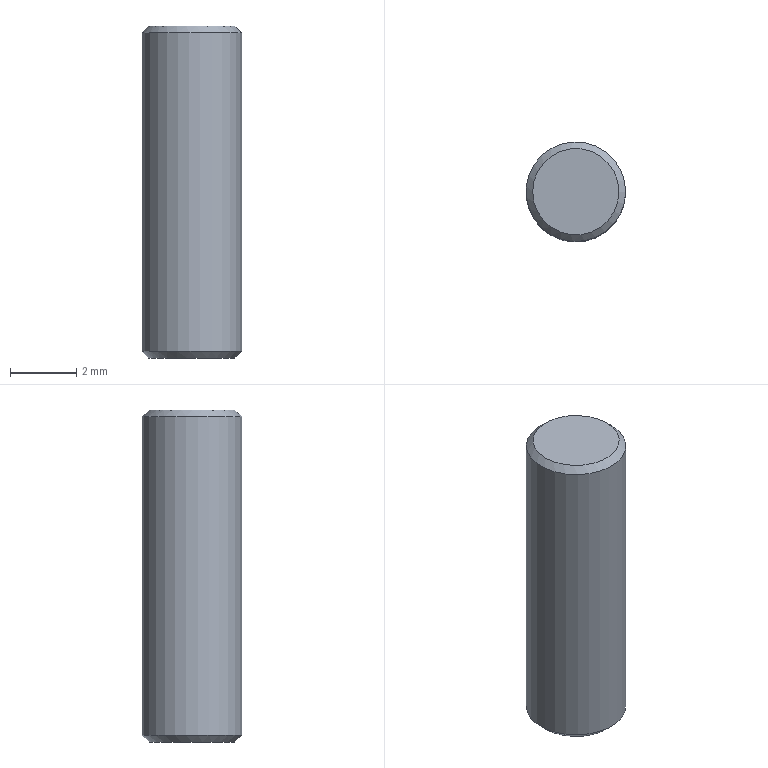Component | NX | GB120-3X10 | 1 solid | 5 faces | box 3 x 3 x 10 mm | volume 70 mm3 | plane 2 | cone 2 | cylinder 1 | commonest cylinder face diameters 3 x1
STEP:
#1=CARTESIAN_POINT('',(0.,0.,0.));
#2=DIRECTION('',(0.,0.,1.));
#3=DIRECTION('',(1.,0.,0.));
#4=AXIS2_PLACEMENT_3D('',#1,#2,#3);
#5=CARTESIAN_POINT('',(-31.5,17.,43.8));
#6=VERTEX_POINT('',#5);
#7=CARTESIAN_POINT('',(-33.,17.,43.8));
#8=DIRECTION('',(0.,0.,-1.));
#9=DIRECTION('',(1.,0.,0.));
#10=AXIS2_PLACEMENT_3D('',#7,#8,#9);
#11=CIRCLE('',#10,1.5);
#12=CARTESIAN_POINT('',(-33.,17.,44.));
#13=DIRECTION('',(0.,0.,-1.));
#14=DIRECTION('',(-1.,0.,0.));
#15=AXIS2_PLACEMENT_3D('',#12,#13,#14);
#16=CYLINDRICAL_SURFACE('',#15,1.5);
#17=CARTESIAN_POINT('',(3.142,0.2));
#18=DIRECTION('',(1.,0.));
#19=VECTOR('',#18,1.);
#20=LINE('',#17,#19);
#21=(GEOMETRIC_REPRESENTATION_CONTEXT(2)PARAMETRIC_REPRESENTATION_CONTEXT()REPRESENTATION_CONTEXT('',''));
#22=DEFINITIONAL_REPRESENTATION('',(#20),#21);
#23=PCURVE('',#16,#22);
#24=CARTESIAN_POINT('',(-33.,17.,44.));
#25=DIRECTION('',(0.,0.,-1.));
#26=DIRECTION('',(-1.,0.,0.));
#27=AXIS2_PLACEMENT_3D('',#24,#25,#26);
#28=CONICAL_SURFACE('',#27,1.3,0.7854);
#29=CARTESIAN_POINT('',(3.142,0.2));
#30=DIRECTION('',(1.,0.));
#31=VECTOR('',#30,1.);
#32=LINE('',#29,#31);
#33=(GEOMETRIC_REPRESENTATION_CONTEXT(2)PARAMETRIC_REPRESENTATION_CONTEXT()REPRESENTATION_CONTEXT('',''));
#34=DEFINITIONAL_REPRESENTATION('',(#32),#33);
#35=PCURVE('',#28,#34);
#36=SURFACE_CURVE('',#11,(#23,#35),.PCURVE_S1.);
#37=EDGE_CURVE('',#6,#6,#36,.T.);
#38=ORIENTED_EDGE('',*,*,#37,.T.);
#39=CARTESIAN_POINT('',(-31.5,17.,34.2));
#40=VERTEX_POINT('',#39);
#41=CARTESIAN_POINT('',(-31.5,17.,43.8));
#42=CARTESIAN_POINT('',(-31.5,17.,34.2));
#43=B_SPLINE_CURVE_WITH_KNOTS('',1,(#41,#42),.UNSPECIFIED.,.F.,.F.,(2,2),(0.2,9.8),.PIECEWISE_BEZIER_KNOTS.);
#44=CARTESIAN_POINT('',(9.425,0.));
#45=DIRECTION('',(0.,1.));
#46=VECTOR('',#45,1.);
#47=LINE('',#44,#46);
#48=(GEOMETRIC_REPRESENTATION_CONTEXT(2)PARAMETRIC_REPRESENTATION_CONTEXT()REPRESENTATION_CONTEXT('',''));
#49=DEFINITIONAL_REPRESENTATION('',(#47),#48);
#50=PCURVE('',#16,#49);
#51=CARTESIAN_POINT('',(3.142,0.));
#52=DIRECTION('',(0.,1.));
#53=VECTOR('',#52,1.);
#54=LINE('',#51,#53);
#55=(GEOMETRIC_REPRESENTATION_CONTEXT(2)PARAMETRIC_REPRESENTATION_CONTEXT()REPRESENTATION_CONTEXT('',''));
#56=DEFINITIONAL_REPRESENTATION('',(#54),#55);
#57=PCURVE('',#16,#56);
#58=SEAM_CURVE('',#43,(#50,#57),.PCURVE_S1.);
#59=EDGE_CURVE('',#6,#40,#58,.T.);
#60=ORIENTED_EDGE('',*,*,#59,.T.);
#61=CARTESIAN_POINT('',(-33.,17.,34.2));
#62=DIRECTION('',(0.,0.,1.));
#63=DIRECTION('',(1.,0.,0.));
#64=AXIS2_PLACEMENT_3D('',#61,#62,#63);
#65=CIRCLE('',#64,1.5);
#66=CARTESIAN_POINT('',(9.425,9.8));
#67=DIRECTION('',(-1.,0.));
#68=VECTOR('',#67,1.);
#69=LINE('',#66,#68);
#70=(GEOMETRIC_REPRESENTATION_CONTEXT(2)PARAMETRIC_REPRESENTATION_CONTEXT()REPRESENTATION_CONTEXT('',''));
#71=DEFINITIONAL_REPRESENTATION('',(#69),#70);
#72=PCURVE('',#16,#71);
#73=CARTESIAN_POINT('',(-33.,17.,34.2));
#74=DIRECTION('',(0.,0.,1.));
#75=DIRECTION('',(1.,0.,0.));
#76=AXIS2_PLACEMENT_3D('',#73,#74,#75);
#77=CONICAL_SURFACE('',#76,1.5,0.7854);
#78=CARTESIAN_POINT('',(0.,0.));
#79=DIRECTION('',(1.,0.));
#80=VECTOR('',#79,1.);
#81=LINE('',#78,#80);
#82=(GEOMETRIC_REPRESENTATION_CONTEXT(2)PARAMETRIC_REPRESENTATION_CONTEXT()REPRESENTATION_CONTEXT('',''));
#83=DEFINITIONAL_REPRESENTATION('',(#81),#82);
#84=PCURVE('',#77,#83);
#85=SURFACE_CURVE('',#65,(#72,#84),.PCURVE_S1.);
#86=EDGE_CURVE('',#40,#40,#85,.T.);
#87=ORIENTED_EDGE('',*,*,#86,.T.);
#88=ORIENTED_EDGE('',*,*,#59,.F.);
#89=EDGE_LOOP('',(#38,#60,#87,#88));
#90=FACE_BOUND('',#89,.T.);
#91=ADVANCED_FACE('',(#90),#16,.T.);
#92=CARTESIAN_POINT('',(-31.7,17.,44.));
#93=VERTEX_POINT('',#92);
#94=CARTESIAN_POINT('',(-33.,17.,44.));
#95=DIRECTION('',(0.,0.,1.));
#96=DIRECTION('',(1.,0.,0.));
#97=AXIS2_PLACEMENT_3D('',#94,#95,#96);
#98=CIRCLE('',#97,1.3);
#99=CARTESIAN_POINT('',(-33.,17.,44.));
#100=DIRECTION('',(0.,0.,1.));
#101=DIRECTION('',(1.,0.,0.));
#102=AXIS2_PLACEMENT_3D('',#99,#100,#101);
#103=PLANE('',#102);
#104=CARTESIAN_POINT('',(0.,0.));
#105=DIRECTION('',(1.,0.));
#106=AXIS2_PLACEMENT_2D('',#104,#105);
#107=CIRCLE('',#106,1.3);
#108=(GEOMETRIC_REPRESENTATION_CONTEXT(2)PARAMETRIC_REPRESENTATION_CONTEXT()REPRESENTATION_CONTEXT('',''));
#109=DEFINITIONAL_REPRESENTATION('',(#107),#108);
#110=PCURVE('',#103,#109);
#111=CARTESIAN_POINT('',(9.425,0.));
#112=DIRECTION('',(-1.,0.));
#113=VECTOR('',#112,1.);
#114=LINE('',#111,#113);
#115=(GEOMETRIC_REPRESENTATION_CONTEXT(2)PARAMETRIC_REPRESENTATION_CONTEXT()REPRESENTATION_CONTEXT('',''));
#116=DEFINITIONAL_REPRESENTATION('',(#114),#115);
#117=PCURVE('',#28,#116);
#118=SURFACE_CURVE('',#98,(#110,#117),.PCURVE_S1.);
#119=EDGE_CURVE('',#93,#93,#118,.T.);
#120=ORIENTED_EDGE('',*,*,#119,.T.);
#121=EDGE_LOOP('',(#120));
#122=FACE_BOUND('',#121,.T.);
#123=ADVANCED_FACE('',(#122),#103,.T.);
#124=CARTESIAN_POINT('',(-31.7,17.,34.));
#125=VERTEX_POINT('',#124);
#126=CARTESIAN_POINT('',(-33.,17.,34.));
#127=DIRECTION('',(0.,0.,-1.));
#128=DIRECTION('',(1.,0.,0.));
#129=AXIS2_PLACEMENT_3D('',#126,#127,#128);
#130=CIRCLE('',#129,1.3);
#131=CARTESIAN_POINT('',(-33.,17.,34.));
#132=DIRECTION('',(0.,0.,1.));
#133=DIRECTION('',(1.,0.,0.));
#134=AXIS2_PLACEMENT_3D('',#131,#132,#133);
#135=PLANE('',#134);
#136=CARTESIAN_POINT('',(1.3,0.));
#137=CARTESIAN_POINT('',(1.3,-2.252));
#138=CARTESIAN_POINT('',(-0.65,-1.126));
#139=CARTESIAN_POINT('',(-2.6,-0.));
#140=CARTESIAN_POINT('',(-0.65,1.126));
#141=CARTESIAN_POINT('',(1.3,2.252));
#142=CARTESIAN_POINT('',(1.3,0.));
#143=(BOUNDED_CURVE()B_SPLINE_CURVE(2,(#136,#137,#138,#139,#140,#141,#142),.UNSPECIFIED.,.T.,.F.)B_SPLINE_CURVE_WITH_KNOTS((1,2,2,2,2,1),(-2.094,0.,2.094,4.189,6.283,8.378),.UNSPECIFIED.)CURVE()GEOMETRIC_REPRESENTATION_ITEM()RATIONAL_B_SPLINE_CURVE((1.,0.5,1.,0.5,1.,0.5,1.))REPRESENTATION_ITEM(''));
#144=(GEOMETRIC_REPRESENTATION_CONTEXT(2)PARAMETRIC_REPRESENTATION_CONTEXT()REPRESENTATION_CONTEXT('',''));
#145=DEFINITIONAL_REPRESENTATION('',(#143),#144);
#146=PCURVE('',#135,#145);
#147=CARTESIAN_POINT('',(6.283,-0.2));
#148=DIRECTION('',(-1.,0.));
#149=VECTOR('',#148,1.);
#150=LINE('',#147,#149);
#151=(GEOMETRIC_REPRESENTATION_CONTEXT(2)PARAMETRIC_REPRESENTATION_CONTEXT()REPRESENTATION_CONTEXT('',''));
#152=DEFINITIONAL_REPRESENTATION('',(#150),#151);
#153=PCURVE('',#77,#152);
#154=SURFACE_CURVE('',#130,(#146,#153),.PCURVE_S1.);
#155=EDGE_CURVE('',#125,#125,#154,.T.);
#156=ORIENTED_EDGE('',*,*,#155,.T.);
#157=EDGE_LOOP('',(#156));
#158=FACE_BOUND('',#157,.T.);
#159=ADVANCED_FACE('',(#158),#135,.F.);
#160=ORIENTED_EDGE('',*,*,#37,.F.);
#161=CARTESIAN_POINT('',(-31.7,17.,44.));
#162=CARTESIAN_POINT('',(-31.5,17.,43.8));
#163=B_SPLINE_CURVE_WITH_KNOTS('',1,(#161,#162),.UNSPECIFIED.,.F.,.F.,(2,2),(0.,0.2828),.PIECEWISE_BEZIER_KNOTS.);
#164=CARTESIAN_POINT('',(3.142,0.));
#165=DIRECTION('',(0.,1.));
#166=VECTOR('',#165,1.);
#167=LINE('',#164,#166);
#168=(GEOMETRIC_REPRESENTATION_CONTEXT(2)PARAMETRIC_REPRESENTATION_CONTEXT()REPRESENTATION_CONTEXT('',''));
#169=DEFINITIONAL_REPRESENTATION('',(#167),#168);
#170=PCURVE('',#28,#169);
#171=CARTESIAN_POINT('',(9.425,0.));
#172=DIRECTION('',(0.,1.));
#173=VECTOR('',#172,1.);
#174=LINE('',#171,#173);
#175=(GEOMETRIC_REPRESENTATION_CONTEXT(2)PARAMETRIC_REPRESENTATION_CONTEXT()REPRESENTATION_CONTEXT('',''));
#176=DEFINITIONAL_REPRESENTATION('',(#174),#175);
#177=PCURVE('',#28,#176);
#178=SEAM_CURVE('',#163,(#170,#177),.PCURVE_S1.);
#179=EDGE_CURVE('',#93,#6,#178,.T.);
#180=ORIENTED_EDGE('',*,*,#179,.F.);
#181=ORIENTED_EDGE('',*,*,#119,.F.);
#182=ORIENTED_EDGE('',*,*,#179,.T.);
#183=EDGE_LOOP('',(#160,#180,#181,#182));
#184=FACE_BOUND('',#183,.T.);
#185=ADVANCED_FACE('',(#184),#28,.T.);
#186=ORIENTED_EDGE('',*,*,#155,.F.);
#187=CARTESIAN_POINT('',(-31.7,17.,34.));
#188=CARTESIAN_POINT('',(-31.5,17.,34.2));
#189=B_SPLINE_CURVE_WITH_KNOTS('',1,(#187,#188),.UNSPECIFIED.,.F.,.F.,(2,2),(-0.2828,0.),.PIECEWISE_BEZIER_KNOTS.);
#190=CARTESIAN_POINT('',(6.283,0.));
#191=DIRECTION('',(0.,1.));
#192=VECTOR('',#191,1.);
#193=LINE('',#190,#192);
#194=(GEOMETRIC_REPRESENTATION_CONTEXT(2)PARAMETRIC_REPRESENTATION_CONTEXT()REPRESENTATION_CONTEXT('',''));
#195=DEFINITIONAL_REPRESENTATION('',(#193),#194);
#196=PCURVE('',#77,#195);
#197=CARTESIAN_POINT('',(0.,0.));
#198=DIRECTION('',(0.,1.));
#199=VECTOR('',#198,1.);
#200=LINE('',#197,#199);
#201=(GEOMETRIC_REPRESENTATION_CONTEXT(2)PARAMETRIC_REPRESENTATION_CONTEXT()REPRESENTATION_CONTEXT('',''));
#202=DEFINITIONAL_REPRESENTATION('',(#200),#201);
#203=PCURVE('',#77,#202);
#204=SEAM_CURVE('',#189,(#196,#203),.PCURVE_S1.);
#205=EDGE_CURVE('',#125,#40,#204,.T.);
#206=ORIENTED_EDGE('',*,*,#205,.T.);
#207=ORIENTED_EDGE('',*,*,#86,.F.);
#208=ORIENTED_EDGE('',*,*,#205,.F.);
#209=EDGE_LOOP('',(#186,#206,#207,#208));
#210=FACE_BOUND('',#209,.T.);
#211=ADVANCED_FACE('',(#210),#77,.T.);
#212=CLOSED_SHELL('',(#91,#123,#159,#185,#211));
#213=MANIFOLD_SOLID_BREP('',#212);
#214=(LENGTH_UNIT()NAMED_UNIT(*)SI_UNIT(.MILLI.,.METRE.));
#215=UNCERTAINTY_MEASURE_WITH_UNIT(LENGTH_MEASURE(0.00001),#214,'','');
#216=(NAMED_UNIT(*)PLANE_ANGLE_UNIT()SI_UNIT($,.RADIAN.));
#217=(NAMED_UNIT(*)SI_UNIT($,.STERADIAN.)SOLID_ANGLE_UNIT());
#218=(GEOMETRIC_REPRESENTATION_CONTEXT(3)GLOBAL_UNCERTAINTY_ASSIGNED_CONTEXT((#215))GLOBAL_UNIT_ASSIGNED_CONTEXT((#214,#216,#217))REPRESENTATION_CONTEXT('',''));
#219=ADVANCED_BREP_SHAPE_REPRESENTATION('',(#4,#213),#218);